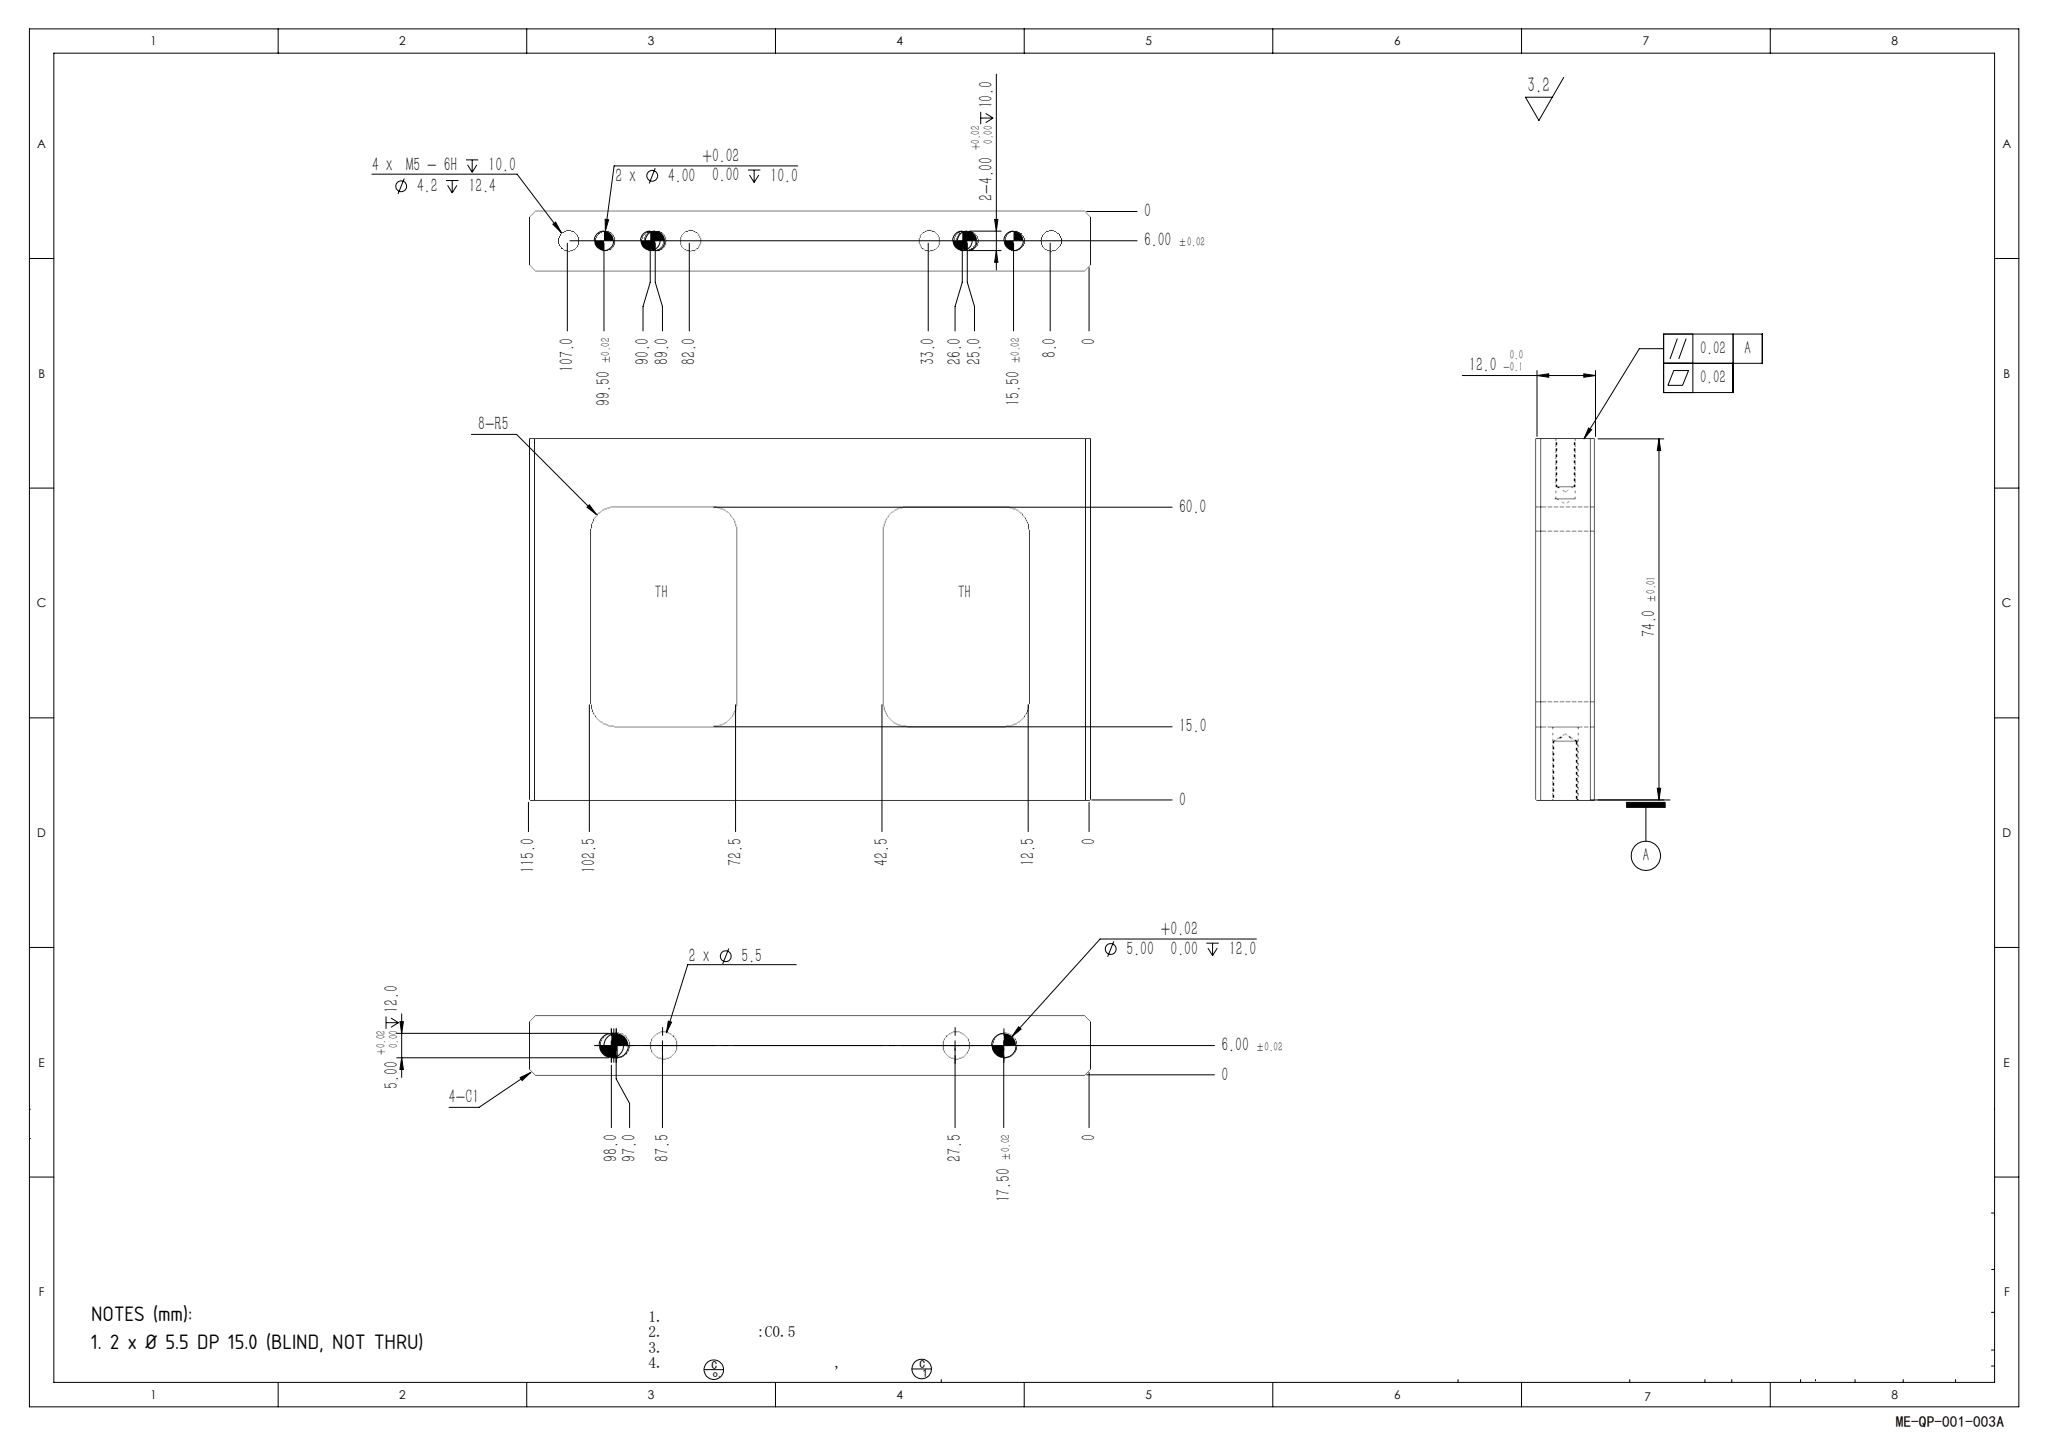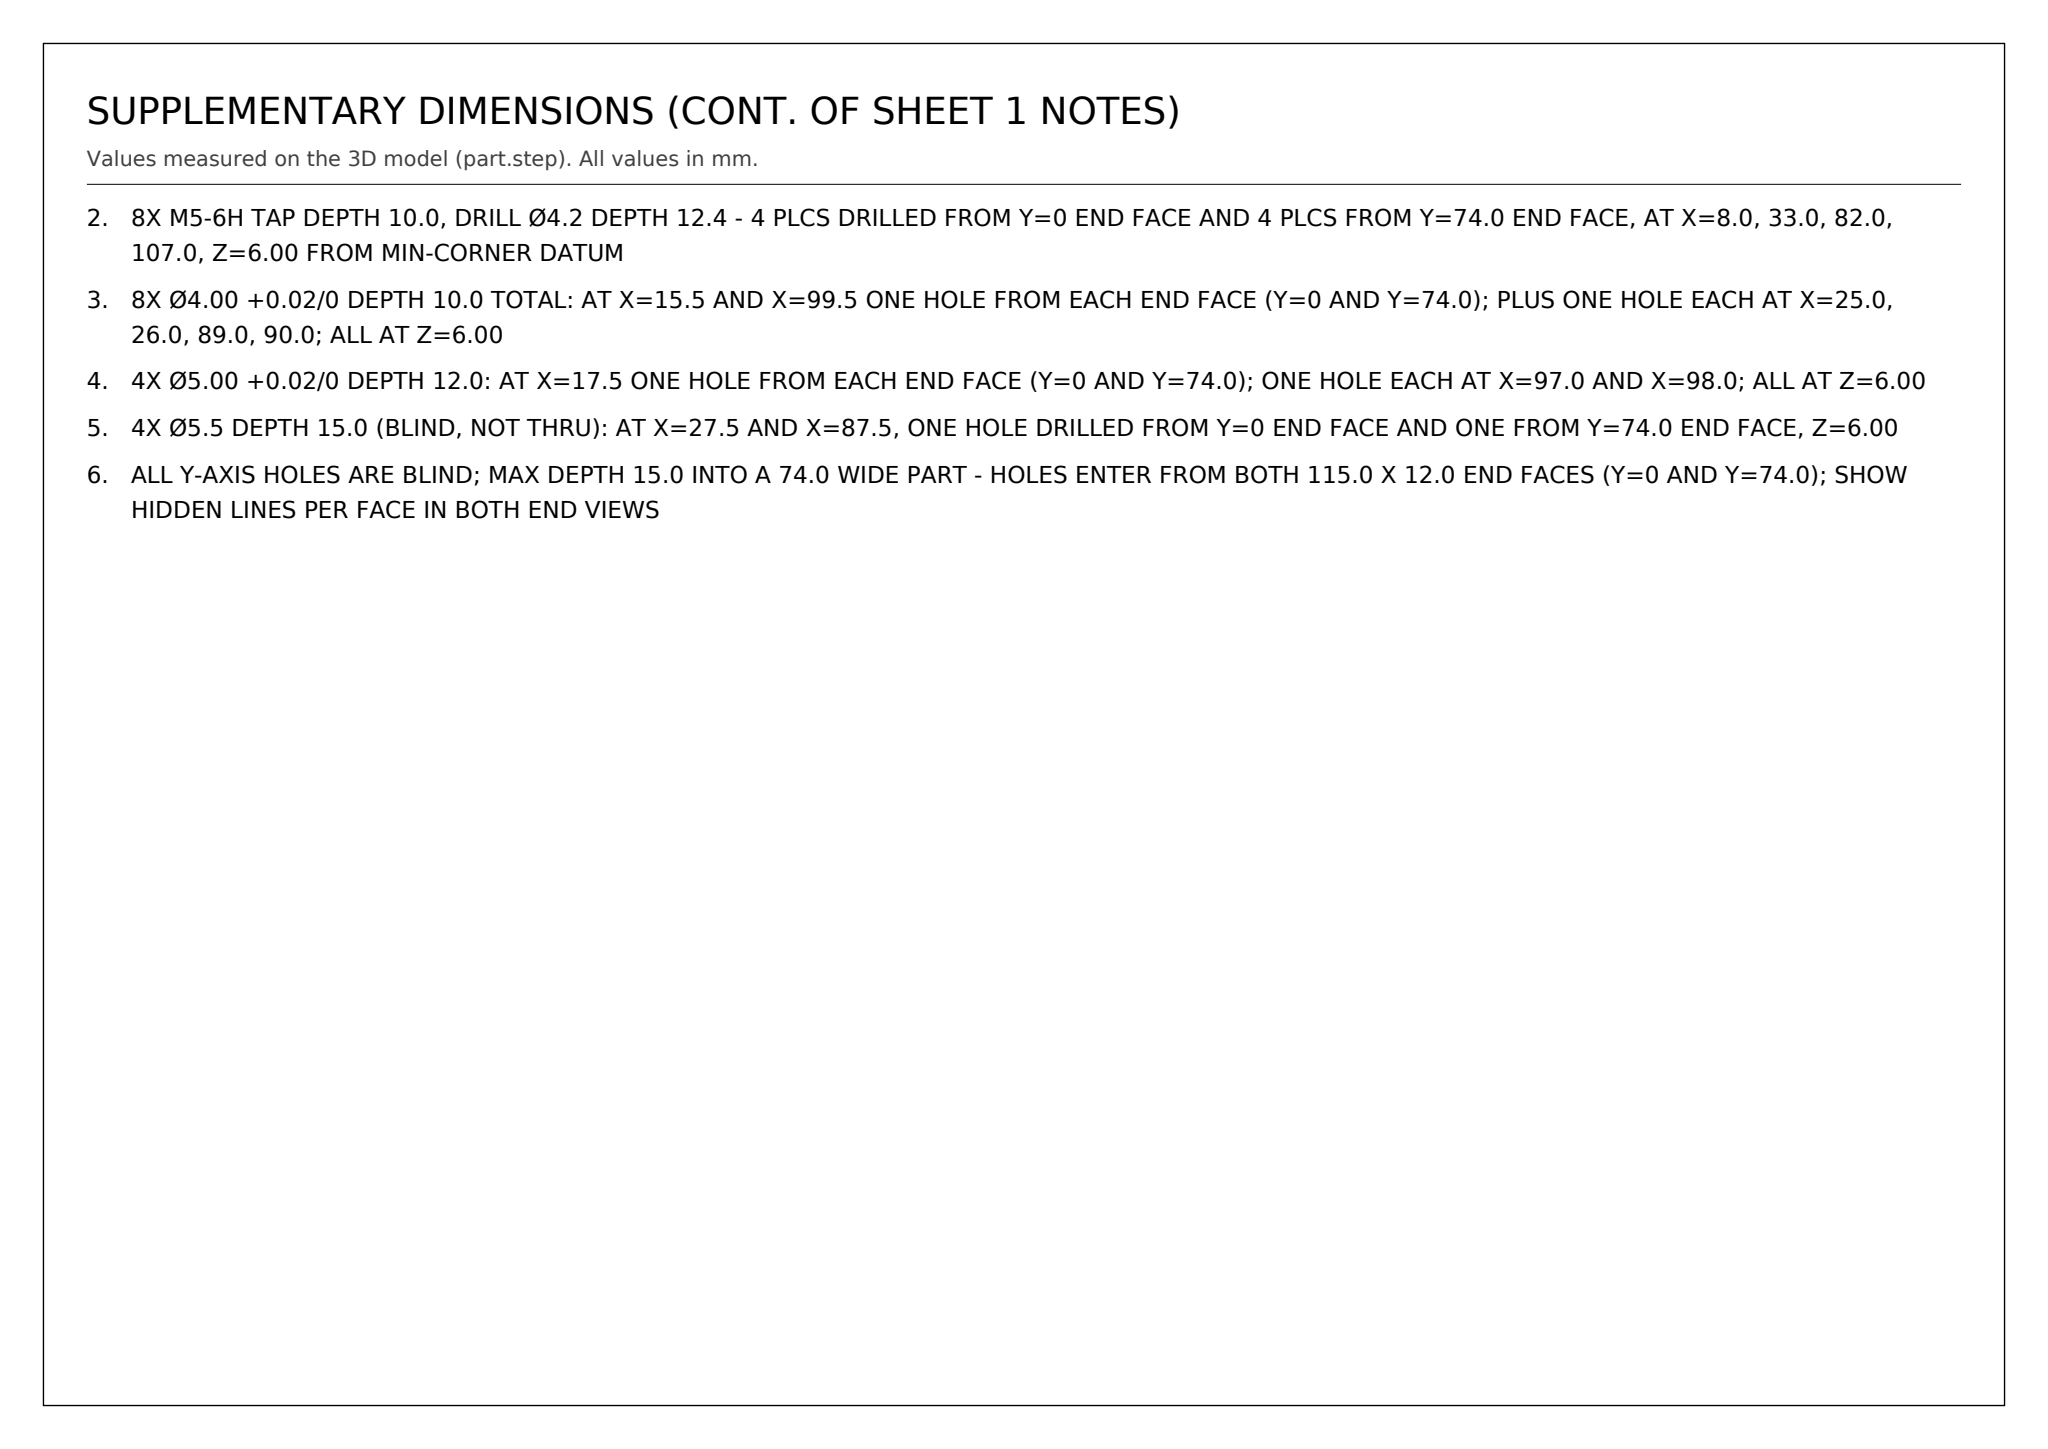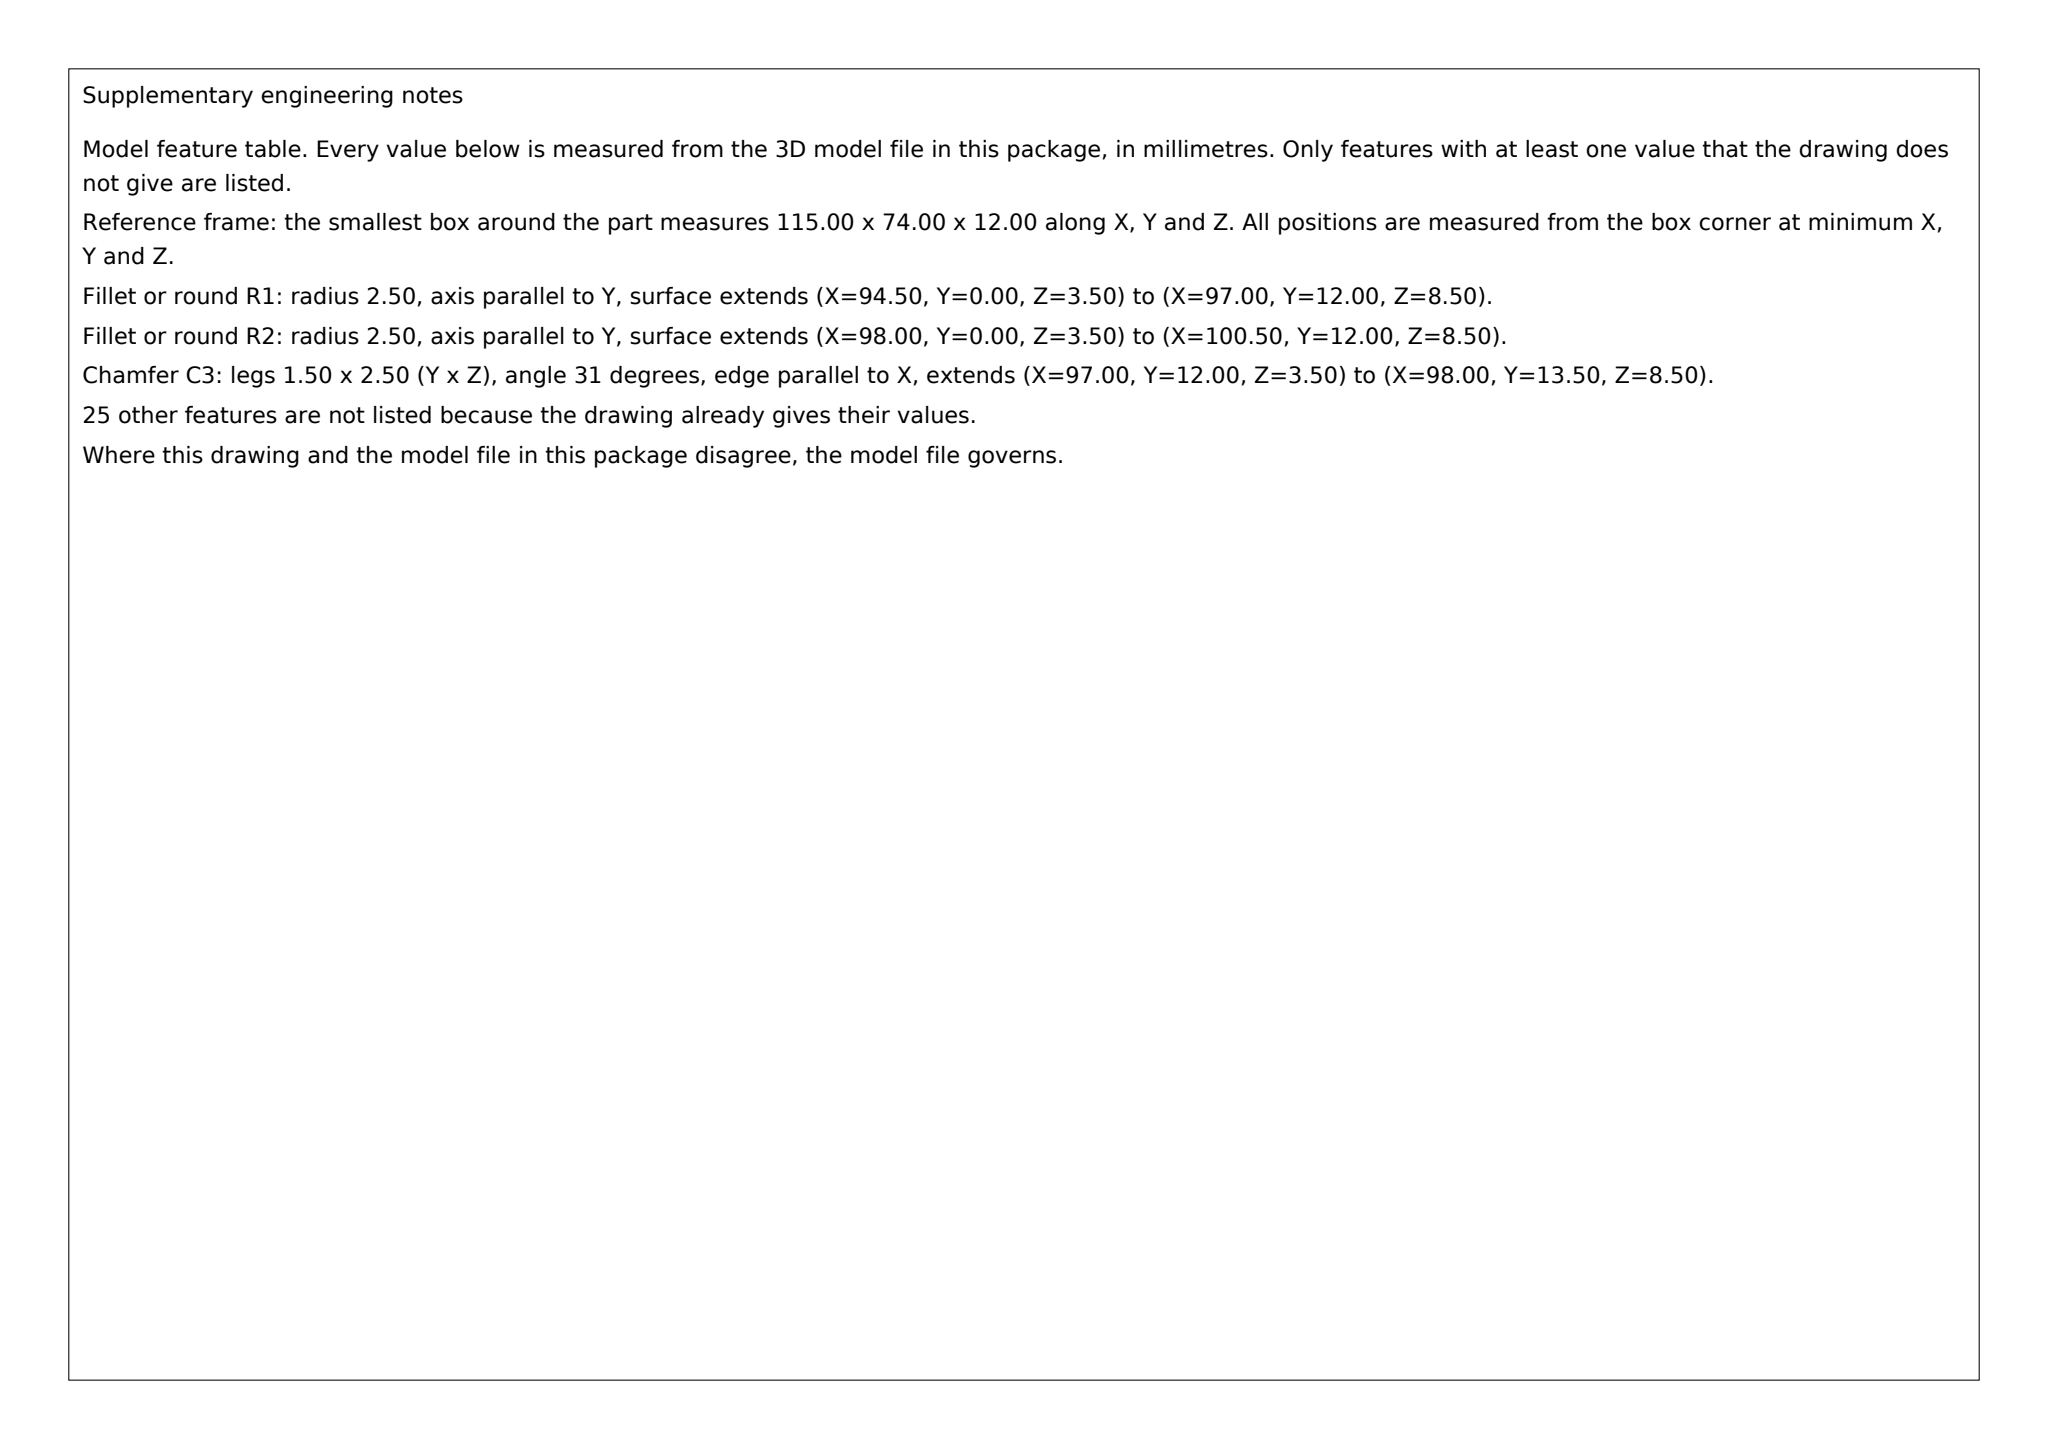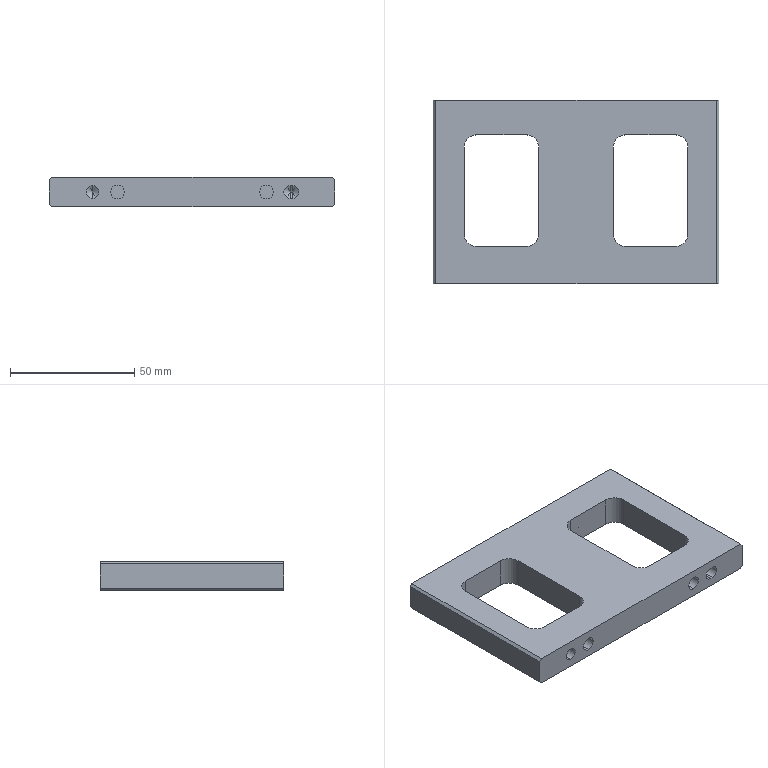Part | SolidWorks | mm | 1 solid | 82 faces | box 115 x 74 x 12 mm | volume 67506 mm3 | cylinder 32 | plane 30 | cone 20 | commonest cylinder face diameters 4 x8 4.2 x8 10 x8 5 x4 5.5 x4
Drawing notes:
2 x Ø 5.5 DP 15.0 (BLIND, NOT THRU) | from the solid: cylinders dia 5.5, axis y, length 15.0 at x=27.5 and x=87.5, z=6.0; part is 74.0 wide in y
8X M5-6H TAP DEPTH 10.0, DRILL Ø4.2 DEPTH 12.4 - 4 PLCS DRILLED FROM Y=0 END FACE AND 4 PLCS FROM Y=74.0 END FACE, AT X=8.0, 33.0, 82.0, 107.0, Z=6.00 FROM MIN-CORNER DATUM | from the solid: cylinders dia 4.2, axis y, pos (x=8.0 / 33.0 / 82.0 / 107.0, z=6.0), length 12.4, count 2 each = 8 total; cones 118deg ref_dia 4.2 count 8
8X Ø4.00 +0.02/0 DEPTH 10.0 TOTAL: AT X=15.5 AND X=99.5 ONE HOLE FROM EACH END FACE (Y=0 AND Y=74.0); PLUS ONE HOLE EACH AT X=25.0, 26.0, 89.0, 90.0; ALL AT Z=6.00 | from the solid: cylinders dia 4.0, axis y, z=6.0, length 10.0: x=15.5 count 2, x=99.5 count 2, x=25.0/26.0/89.0/90.0 count 1 each = 8 total; cones 118deg ref_dia 4.0 count 8
4X Ø5.00 +0.02/0 DEPTH 12.0: AT X=17.5 ONE HOLE FROM EACH END FACE (Y=0 AND Y=74.0); ONE HOLE EACH AT X=97.0 AND X=98.0; ALL AT Z=6.00 | from the solid: cylinders dia 5.0, axis y, z=6.0, length 12.0: x=17.5 count 2, x=97.0 count 1, x=98.0 count 1; cones 118deg ref_dia 5.0 count 4
4X Ø5.5 DEPTH 15.0 (BLIND, NOT THRU): AT X=27.5 AND X=87.5, ONE HOLE DRILLED FROM Y=0 END FACE AND ONE FROM Y=74.0 END FACE, Z=6.00 | from the solid: cylinders dia 5.5, axis y, pos (x=27.5 and x=87.5, z=6.0), length 15.0, count 2 each = 4 total
ALL Y-AXIS HOLES ARE BLIND; MAX DEPTH 15.0 INTO A 74.0 WIDE PART - HOLES ENTER FROM BOTH 115.0 X 12.0 END FACES (Y=0 AND Y=74.0); SHOW HIDDEN LINES PER FACE IN BOTH END VIEWS | from the solid: bbox_xyz 115.0 x 74.0 x 12.0; axis_planes y 0.0 and y 74.0; all y-axis cylinder lengths <= 15.0